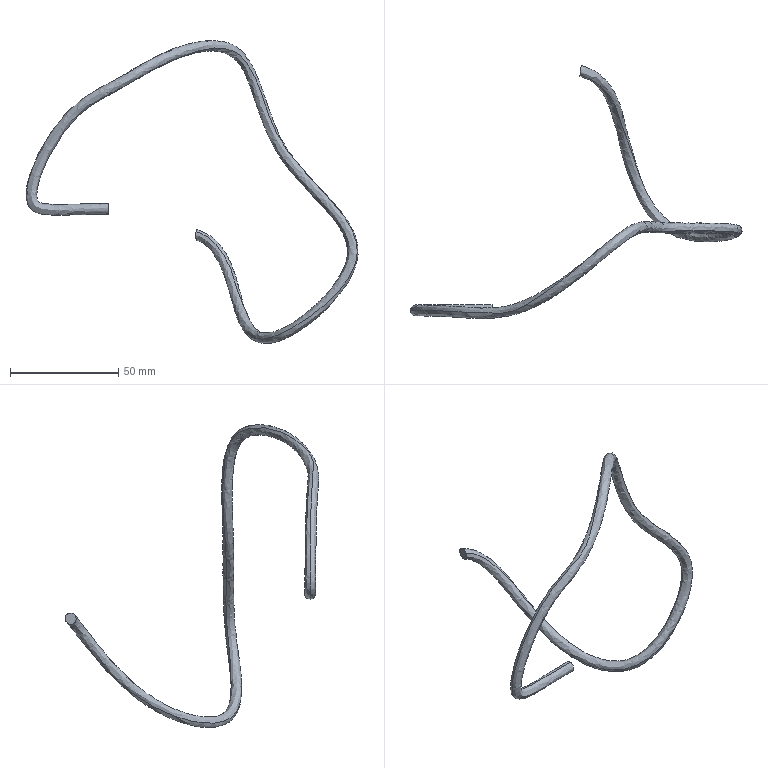Component | SolidWorks | Wire-1 | 1 solid | 4 faces | volume 8681 mm3 | spline 2 | plane 2 | material 45